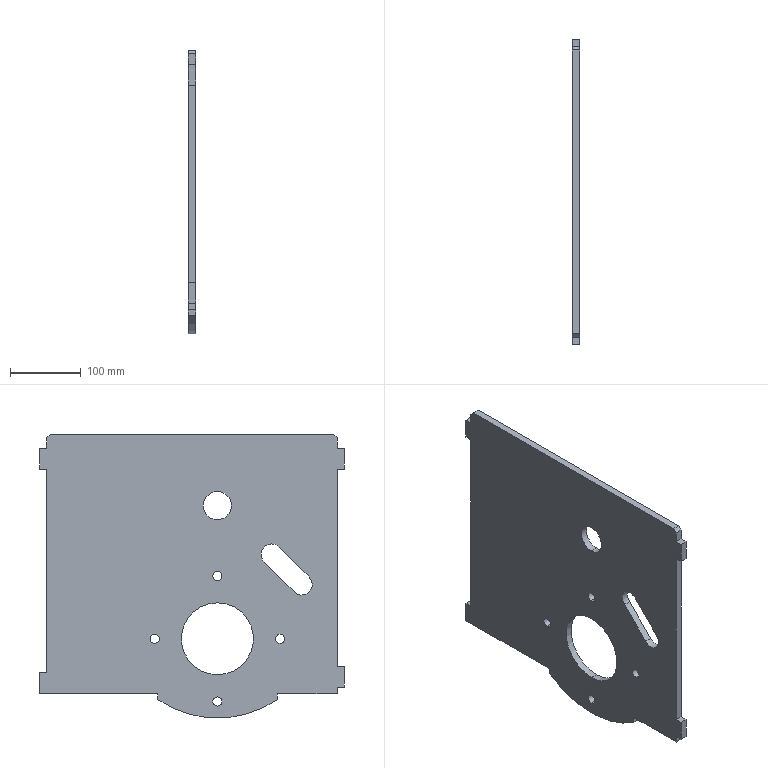Component | SolidWorks | BrakeMountingPlate-1 | 1 solid | 43 faces | box 10 x 432 x 402.5 mm | volume 1447157 mm3 | plane 27 | cylinder 16 | commonest cylinder face diameters 13.1 x8 30 x3 102 x2 40 x2 298.213 x1 | material Q235
build123d program:
from build123d import *

# Parameters (mm, degrees)
SKETCH1_R           = 51
SKETCH1_R_2         = 20
BOSS_EXTRUDE1_DEPTH = 10


with BuildPart() as part:
    # Sketch1 → Boss-Extrude1 (new body)
    with BuildSketch(Plane(origin=(0, 0, 0), x_dir=(1, 0, 0), z_dir=(0, 1, 0))):
        with BuildLine():
            Line((307.81, 53.072), (307.81, 61.072))
            Line((307.81, 61.072), (140.368, 61.072))
            Line((140.368, 61.072), (140.368, 91.072))
            Line((140.368, 91.072), (150.368, 91.072))
            Line((150.368, 91.072), (150.368, 379.572))
            Line((150.368, 379.572), (140.368, 379.572))
            Line((140.368, 379.572), (140.368, 409.072))
            Line((140.368, 409.072), (150.368, 409.072))
            Line((150.368, 409.072), (150.368, 424.072))
            Line((150.368, 424.072), (155.368, 429.072))
            Line((155.368, 429.072), (557.368, 429.072))
            Line((557.368, 429.072), (562.368, 424.072))
            Line((562.368, 424.072), (562.368, 409.072))
            Line((562.368, 409.072), (572.368, 409.072))
            Line((572.368, 409.072), (572.368, 379.572))
            Line((572.368, 379.572), (562.368, 379.572))
            Line((562.368, 379.572), (562.368, 100.072))
            Line((562.368, 100.072), (572.368, 100.072))
            Line((572.368, 100.072), (572.368, 70.572))
            Line((572.368, 70.572), (562.368, 70.572))
            Line((562.368, 70.572), (562.368, 61.072))
            Line((562.368, 61.072), (477.521, 61.072))
            Line((477.521, 61.072), (477.521, 53.072))
            ThreePointArc((477.521, 53.072), (392.666, 26.571), (307.81, 53.072))
        make_face()
        with Locations(Location((392.368, 139.072, 0), (0, 0, 270))):
            Circle(SKETCH1_R, mode=Mode.SUBTRACT)
        with Locations(Location((392.368, 327.972, 0), (0, 0, 270))):
            Circle(SKETCH1_R_2, mode=Mode.SUBTRACT)
        with BuildLine():
            ThreePointArc((479.978, 269.108), (458.765, 269.108), (458.765, 247.895))
            Line((458.765, 247.895), (501.192, 205.469))
            ThreePointArc((501.192, 205.469), (522.405, 205.469), (522.405, 226.682))
            Line((522.405, 226.682), (479.978, 269.108))
        make_face(mode=Mode.SUBTRACT)
        with BuildLine():
            ThreePointArc((396.999, 223.34), (396.999, 232.603), (387.736, 232.603))
            ThreePointArc((387.736, 232.603), (387.736, 223.34), (396.999, 223.34))
        make_face(mode=Mode.SUBTRACT)
        with BuildLine():
            ThreePointArc((485.899, 134.44), (485.899, 143.703), (476.636, 143.703))
            ThreePointArc((476.636, 143.703), (476.636, 134.44), (485.899, 134.44))
        make_face(mode=Mode.SUBTRACT)
        with BuildLine():
            ThreePointArc((396.999, 45.54), (396.999, 54.803), (387.736, 54.803))
            ThreePointArc((387.736, 54.803), (387.736, 45.54), (396.999, 45.54))
        make_face(mode=Mode.SUBTRACT)
        with BuildLine():
            ThreePointArc((308.099, 134.44), (308.099, 143.703), (298.836, 143.703))
            ThreePointArc((298.836, 143.703), (298.836, 134.44), (308.099, 134.44))
        make_face(mode=Mode.SUBTRACT)
    extrude(amount=BOSS_EXTRUDE1_DEPTH)


solid = part.part

# Placed as in the assembly
solid = solid.moved(Location((-460.054, -14.958, 2306.634), (180, 0, 90)))